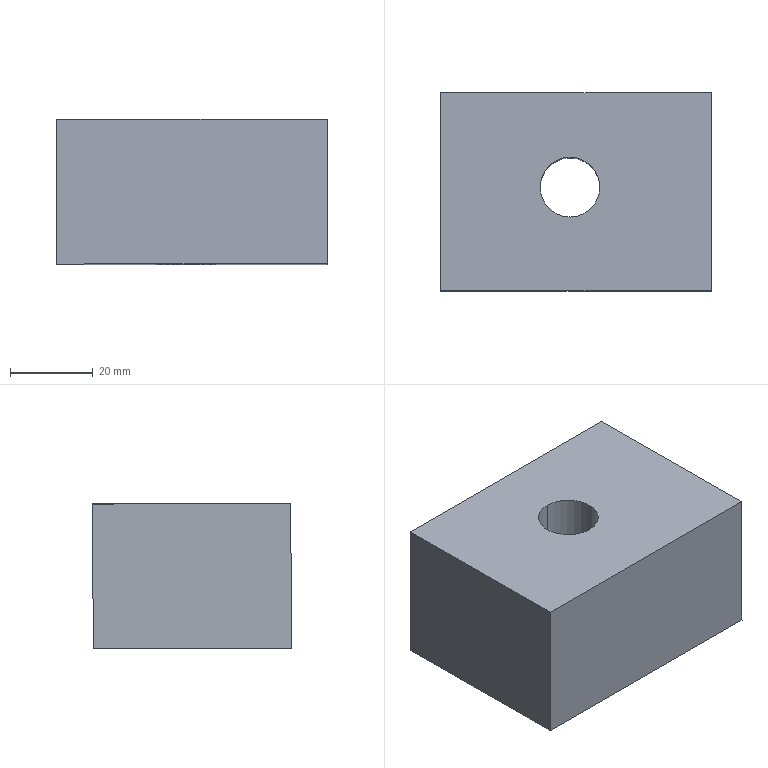Component | SolidWorks | RehabilitationChair-18-17-1 | 1 solid | 8 faces | box 65.51 x 48.07 x 35.2 mm | volume 104150 mm3 | plane 6 | cylinder 2 | commonest cylinder face diameters 14.46 x2
STEP:
#1=COLOUR_RGB('',0.7922,0.8196,0.9333);
#2=FILL_AREA_STYLE_COLOUR('',#1);
#3=FILL_AREA_STYLE('',(#2));
#4=SURFACE_STYLE_FILL_AREA(#3);
#5=SURFACE_SIDE_STYLE('',(#4));
#6=SURFACE_STYLE_USAGE(.BOTH.,#5);
#7=PRESENTATION_STYLE_ASSIGNMENT((#6));
#8=CARTESIAN_POINT('',(15.972,7.157,11.065));
#9=VERTEX_POINT('',#8);
#10=CARTESIAN_POINT('',(15.972,7.726,11.063));
#11=VERTEX_POINT('',#10);
#12=CARTESIAN_POINT('',(15.972,7.442,11.064));
#13=DIRECTION('',(-0.0003323,0.003798,1.));
#14=DIRECTION('',(0.,-1.,0.003798));
#15=AXIS2_PLACEMENT_3D('',#12,#13,#14);
#16=CIRCLE('',#15,0.2846);
#17=EDGE_CURVE('',#9,#11,#16,.T.);
#18=ORIENTED_EDGE('',*,*,#17,.F.);
#19=CARTESIAN_POINT('',(15.971,7.162,12.443));
#20=VERTEX_POINT('',#19);
#21=CARTESIAN_POINT('',(15.971,7.162,12.422));
#22=DIRECTION('',(-0.0003323,0.003798,1.));
#23=VECTOR('',#22,39.37);
#24=LINE('',#21,#23);
#25=EDGE_CURVE('',#9,#20,#24,.T.);
#26=ORIENTED_EDGE('',*,*,#25,.T.);
#27=CARTESIAN_POINT('',(15.971,7.732,12.441));
#28=VERTEX_POINT('',#27);
#29=CARTESIAN_POINT('',(15.971,7.447,12.442));
#30=DIRECTION('',(-0.0003323,0.003798,1.));
#31=DIRECTION('',(0.,1.,-0.003798));
#32=AXIS2_PLACEMENT_3D('',#29,#30,#31);
#33=CIRCLE('',#32,0.2846);
#34=EDGE_CURVE('',#20,#28,#33,.T.);
#35=ORIENTED_EDGE('',*,*,#34,.T.);
#36=CARTESIAN_POINT('',(15.971,7.732,12.42));
#37=DIRECTION('',(-0.0003323,0.003798,1.));
#38=VECTOR('',#37,39.37);
#39=LINE('',#36,#38);
#40=EDGE_CURVE('',#11,#28,#39,.T.);
#41=ORIENTED_EDGE('',*,*,#40,.F.);
#42=EDGE_LOOP('',(#18,#26,#35,#41));
#43=FACE_OUTER_BOUND('',#42,.T.);
#44=CARTESIAN_POINT('',(15.971,7.447,12.421));
#45=DIRECTION('',(-0.0003323,0.003798,1.));
#46=DIRECTION('',(0.,1.,-0.003798));
#47=AXIS2_PLACEMENT_3D('',#44,#45,#46);
#48=CYLINDRICAL_SURFACE('',#47,0.2846);
#49=ADVANCED_FACE('',(#43),#48,.F.);
#50=CARTESIAN_POINT('',(17.317,8.348,12.439));
#51=VERTEX_POINT('',#50);
#52=CARTESIAN_POINT('',(14.739,8.348,12.438));
#53=VERTEX_POINT('',#52);
#54=CARTESIAN_POINT('',(14.739,8.348,12.438));
#55=DIRECTION('',(-1.,-0.00000126,-0.0003323));
#56=VECTOR('',#55,39.37);
#57=LINE('',#54,#56);
#58=EDGE_CURVE('',#51,#53,#57,.T.);
#59=ORIENTED_EDGE('',*,*,#58,.T.);
#60=CARTESIAN_POINT('',(14.739,6.461,12.445));
#61=VERTEX_POINT('',#60);
#62=CARTESIAN_POINT('',(14.739,8.348,12.438));
#63=DIRECTION('',(0.,-1.,0.003798));
#64=VECTOR('',#63,39.37);
#65=LINE('',#62,#64);
#66=EDGE_CURVE('',#53,#61,#65,.T.);
#67=ORIENTED_EDGE('',*,*,#66,.T.);
#68=CARTESIAN_POINT('',(17.317,6.461,12.446));
#69=VERTEX_POINT('',#68);
#70=CARTESIAN_POINT('',(14.739,6.461,12.445));
#71=DIRECTION('',(1.,0.00000126,0.0003323));
#72=VECTOR('',#71,39.37);
#73=LINE('',#70,#72);
#74=EDGE_CURVE('',#61,#69,#73,.T.);
#75=ORIENTED_EDGE('',*,*,#74,.T.);
#76=CARTESIAN_POINT('',(17.317,8.348,12.439));
#77=DIRECTION('',(0.,1.,-0.003798));
#78=VECTOR('',#77,39.37);
#79=LINE('',#76,#78);
#80=EDGE_CURVE('',#69,#51,#79,.T.);
#81=ORIENTED_EDGE('',*,*,#80,.T.);
#82=EDGE_LOOP('',(#59,#67,#75,#81));
#83=FACE_OUTER_BOUND('',#82,.T.);
#84=CARTESIAN_POINT('',(15.971,7.447,12.442));
#85=DIRECTION('',(-0.0003323,0.003798,1.));
#86=DIRECTION('',(0.,1.,-0.003798));
#87=AXIS2_PLACEMENT_3D('',#84,#85,#86);
#88=CIRCLE('',#87,0.2846);
#89=EDGE_CURVE('',#28,#20,#88,.T.);
#90=ORIENTED_EDGE('',*,*,#89,.F.);
#91=ORIENTED_EDGE('',*,*,#34,.F.);
#92=EDGE_LOOP('',(#90,#91));
#93=FACE_BOUND('',#92,.T.);
#94=CARTESIAN_POINT('',(14.739,7.321,12.442));
#95=DIRECTION('',(0.0003323,-0.003798,-1.));
#96=DIRECTION('',(0.,1.,-0.003798));
#97=AXIS2_PLACEMENT_3D('',#94,#95,#96);
#98=PLANE('',#97);
#99=ADVANCED_FACE('',(#83,#93),#98,.F.);
#100=ORIENTED_EDGE('',*,*,#25,.F.);
#101=CARTESIAN_POINT('',(15.972,7.442,11.064));
#102=DIRECTION('',(-0.0003323,0.003798,1.));
#103=DIRECTION('',(0.,-1.,0.003798));
#104=AXIS2_PLACEMENT_3D('',#101,#102,#103);
#105=CIRCLE('',#104,0.2846);
#106=EDGE_CURVE('',#11,#9,#105,.T.);
#107=ORIENTED_EDGE('',*,*,#106,.F.);
#108=ORIENTED_EDGE('',*,*,#40,.T.);
#109=ORIENTED_EDGE('',*,*,#89,.T.);
#110=EDGE_LOOP('',(#100,#107,#108,#109));
#111=FACE_OUTER_BOUND('',#110,.T.);
#112=CARTESIAN_POINT('',(15.971,7.447,12.421));
#113=DIRECTION('',(-0.0003323,0.003798,1.));
#114=DIRECTION('',(0.,1.,-0.003798));
#115=AXIS2_PLACEMENT_3D('',#112,#113,#114);
#116=CYLINDRICAL_SURFACE('',#115,0.2846);
#117=ADVANCED_FACE('',(#111),#116,.F.);
#118=ORIENTED_EDGE('',*,*,#66,.F.);
#119=CARTESIAN_POINT('',(14.739,8.343,11.06));
#120=VERTEX_POINT('',#119);
#121=CARTESIAN_POINT('',(14.739,8.343,11.06));
#122=DIRECTION('',(-0.0003323,0.003798,1.));
#123=VECTOR('',#122,39.37);
#124=LINE('',#121,#123);
#125=EDGE_CURVE('',#120,#53,#124,.T.);
#126=ORIENTED_EDGE('',*,*,#125,.F.);
#127=CARTESIAN_POINT('',(14.739,6.456,11.068));
#128=VERTEX_POINT('',#127);
#129=CARTESIAN_POINT('',(14.739,8.343,11.06));
#130=DIRECTION('',(0.,-1.,0.003798));
#131=VECTOR('',#130,39.37);
#132=LINE('',#129,#131);
#133=EDGE_CURVE('',#120,#128,#132,.T.);
#134=ORIENTED_EDGE('',*,*,#133,.T.);
#135=CARTESIAN_POINT('',(14.739,6.456,11.068));
#136=DIRECTION('',(-0.0003323,0.003798,1.));
#137=VECTOR('',#136,39.37);
#138=LINE('',#135,#137);
#139=EDGE_CURVE('',#128,#61,#138,.T.);
#140=ORIENTED_EDGE('',*,*,#139,.T.);
#141=EDGE_LOOP('',(#118,#126,#134,#140));
#142=FACE_OUTER_BOUND('',#141,.T.);
#143=CARTESIAN_POINT('',(14.739,8.343,11.06));
#144=DIRECTION('',(1.,0.00000126,0.0003323));
#145=DIRECTION('',(-0.0003323,0.,1.));
#146=AXIS2_PLACEMENT_3D('',#143,#144,#145);
#147=PLANE('',#146);
#148=ADVANCED_FACE('',(#142),#147,.F.);
#149=ORIENTED_EDGE('',*,*,#58,.F.);
#150=CARTESIAN_POINT('',(17.318,8.343,11.061));
#151=VERTEX_POINT('',#150);
#152=CARTESIAN_POINT('',(17.318,8.343,11.061));
#153=DIRECTION('',(-0.0003323,0.003798,1.));
#154=VECTOR('',#153,39.37);
#155=LINE('',#152,#154);
#156=EDGE_CURVE('',#151,#51,#155,.T.);
#157=ORIENTED_EDGE('',*,*,#156,.F.);
#158=CARTESIAN_POINT('',(14.739,8.343,11.06));
#159=DIRECTION('',(-1.,-0.00000126,-0.0003323));
#160=VECTOR('',#159,39.37);
#161=LINE('',#158,#160);
#162=EDGE_CURVE('',#151,#120,#161,.T.);
#163=ORIENTED_EDGE('',*,*,#162,.T.);
#164=ORIENTED_EDGE('',*,*,#125,.T.);
#165=EDGE_LOOP('',(#149,#157,#163,#164));
#166=FACE_OUTER_BOUND('',#165,.T.);
#167=CARTESIAN_POINT('',(14.739,8.343,11.06));
#168=DIRECTION('',(-0.,-1.,0.003798));
#169=DIRECTION('',(0.,0.003798,1.));
#170=AXIS2_PLACEMENT_3D('',#167,#168,#169);
#171=PLANE('',#170);
#172=ADVANCED_FACE('',(#166),#171,.F.);
#173=ORIENTED_EDGE('',*,*,#106,.T.);
#174=ORIENTED_EDGE('',*,*,#17,.T.);
#175=EDGE_LOOP('',(#173,#174));
#176=FACE_BOUND('',#175,.T.);
#177=ORIENTED_EDGE('',*,*,#133,.F.);
#178=ORIENTED_EDGE('',*,*,#162,.F.);
#179=CARTESIAN_POINT('',(17.318,6.456,11.068));
#180=VERTEX_POINT('',#179);
#181=CARTESIAN_POINT('',(17.318,8.343,11.061));
#182=DIRECTION('',(0.,1.,-0.003798));
#183=VECTOR('',#182,39.37);
#184=LINE('',#181,#183);
#185=EDGE_CURVE('',#180,#151,#184,.T.);
#186=ORIENTED_EDGE('',*,*,#185,.F.);
#187=CARTESIAN_POINT('',(14.739,6.456,11.068));
#188=DIRECTION('',(1.,0.00000126,0.0003323));
#189=VECTOR('',#188,39.37);
#190=LINE('',#187,#189);
#191=EDGE_CURVE('',#128,#180,#190,.T.);
#192=ORIENTED_EDGE('',*,*,#191,.F.);
#193=EDGE_LOOP('',(#177,#178,#186,#192));
#194=FACE_OUTER_BOUND('',#193,.T.);
#195=CARTESIAN_POINT('',(-0.003684,0.04211,11.087));
#196=DIRECTION('',(0.0003323,-0.003798,-1.));
#197=DIRECTION('',(0.,-1.,0.003798));
#198=AXIS2_PLACEMENT_3D('',#195,#196,#197);
#199=PLANE('',#198);
#200=ADVANCED_FACE('',(#176,#194),#199,.T.);
#201=ORIENTED_EDGE('',*,*,#74,.F.);
#202=ORIENTED_EDGE('',*,*,#139,.F.);
#203=ORIENTED_EDGE('',*,*,#191,.T.);
#204=CARTESIAN_POINT('',(17.318,6.456,11.068));
#205=DIRECTION('',(-0.0003323,0.003798,1.));
#206=VECTOR('',#205,39.37);
#207=LINE('',#204,#206);
#208=EDGE_CURVE('',#180,#69,#207,.T.);
#209=ORIENTED_EDGE('',*,*,#208,.T.);
#210=EDGE_LOOP('',(#201,#202,#203,#209));
#211=FACE_OUTER_BOUND('',#210,.T.);
#212=CARTESIAN_POINT('',(14.739,6.456,11.068));
#213=DIRECTION('',(0.,1.,-0.003798));
#214=DIRECTION('',(0.,-0.003798,-1.));
#215=AXIS2_PLACEMENT_3D('',#212,#213,#214);
#216=PLANE('',#215);
#217=ADVANCED_FACE('',(#211),#216,.F.);
#218=ORIENTED_EDGE('',*,*,#80,.F.);
#219=ORIENTED_EDGE('',*,*,#208,.F.);
#220=ORIENTED_EDGE('',*,*,#185,.T.);
#221=ORIENTED_EDGE('',*,*,#156,.T.);
#222=EDGE_LOOP('',(#218,#219,#220,#221));
#223=FACE_OUTER_BOUND('',#222,.T.);
#224=CARTESIAN_POINT('',(17.318,8.343,11.061));
#225=DIRECTION('',(-1.,-0.00000126,-0.0003323));
#226=DIRECTION('',(0.0003323,0.,-1.));
#227=AXIS2_PLACEMENT_3D('',#224,#225,#226);
#228=PLANE('',#227);
#229=ADVANCED_FACE('',(#223),#228,.F.);
#230=CLOSED_SHELL('',(#49,#99,#117,#148,#172,#200,#217,#229));
#231=MANIFOLD_SOLID_BREP('',#230);
#232=STYLED_ITEM('',(#7),#231);
#233=PRESENTATION_LAYER_ASSIGNMENT('','',(#232));
#234=CARTESIAN_POINT('',(0.,0.,0.));
#235=DIRECTION('',(0.,0.,1.));
#236=DIRECTION('',(1.,0.,0.));
#237=AXIS2_PLACEMENT_3D('',#234,#235,#236);
#238=(LENGTH_UNIT()NAMED_UNIT(*)SI_UNIT($,.METRE.));
#239=LENGTH_MEASURE_WITH_UNIT(LENGTH_MEASURE(0.0254),#238);
#240=DIMENSIONAL_EXPONENTS(1.,0.,0.,0.,0.,0.,0.);
#241=(CONVERSION_BASED_UNIT('',#239)LENGTH_UNIT()NAMED_UNIT(#240));
#242=UNCERTAINTY_MEASURE_WITH_UNIT(LENGTH_MEASURE(0.00001),#241,'','');
#243=(NAMED_UNIT(*)PLANE_ANGLE_UNIT()SI_UNIT($,.RADIAN.));
#244=(NAMED_UNIT(*)SI_UNIT($,.STERADIAN.)SOLID_ANGLE_UNIT());
#245=(GEOMETRIC_REPRESENTATION_CONTEXT(3)GLOBAL_UNCERTAINTY_ASSIGNED_CONTEXT((#242))GLOBAL_UNIT_ASSIGNED_CONTEXT((#241,#243,#244))REPRESENTATION_CONTEXT('',''));
#246=ADVANCED_BREP_SHAPE_REPRESENTATION('',(#231,#237),#245);
#247=(LENGTH_UNIT()NAMED_UNIT(*)SI_UNIT($,.METRE.));
#248=LENGTH_MEASURE_WITH_UNIT(LENGTH_MEASURE(0.0254),#247);
#249=DIMENSIONAL_EXPONENTS(1.,0.,0.,0.,0.,0.,0.);
#250=(CONVERSION_BASED_UNIT('',#248)LENGTH_UNIT()NAMED_UNIT(#249));
#251=UNCERTAINTY_MEASURE_WITH_UNIT(LENGTH_MEASURE(0.00001),#250,'','');
#252=(NAMED_UNIT(*)PLANE_ANGLE_UNIT()SI_UNIT($,.RADIAN.));
#253=(NAMED_UNIT(*)SI_UNIT($,.STERADIAN.)SOLID_ANGLE_UNIT());
#254=(GEOMETRIC_REPRESENTATION_CONTEXT(3)GLOBAL_UNCERTAINTY_ASSIGNED_CONTEXT((#251))GLOBAL_UNIT_ASSIGNED_CONTEXT((#250,#252,#253))REPRESENTATION_CONTEXT('',''));
#255=MECHANICAL_DESIGN_GEOMETRIC_PRESENTATION_REPRESENTATION('',(#232),#254);